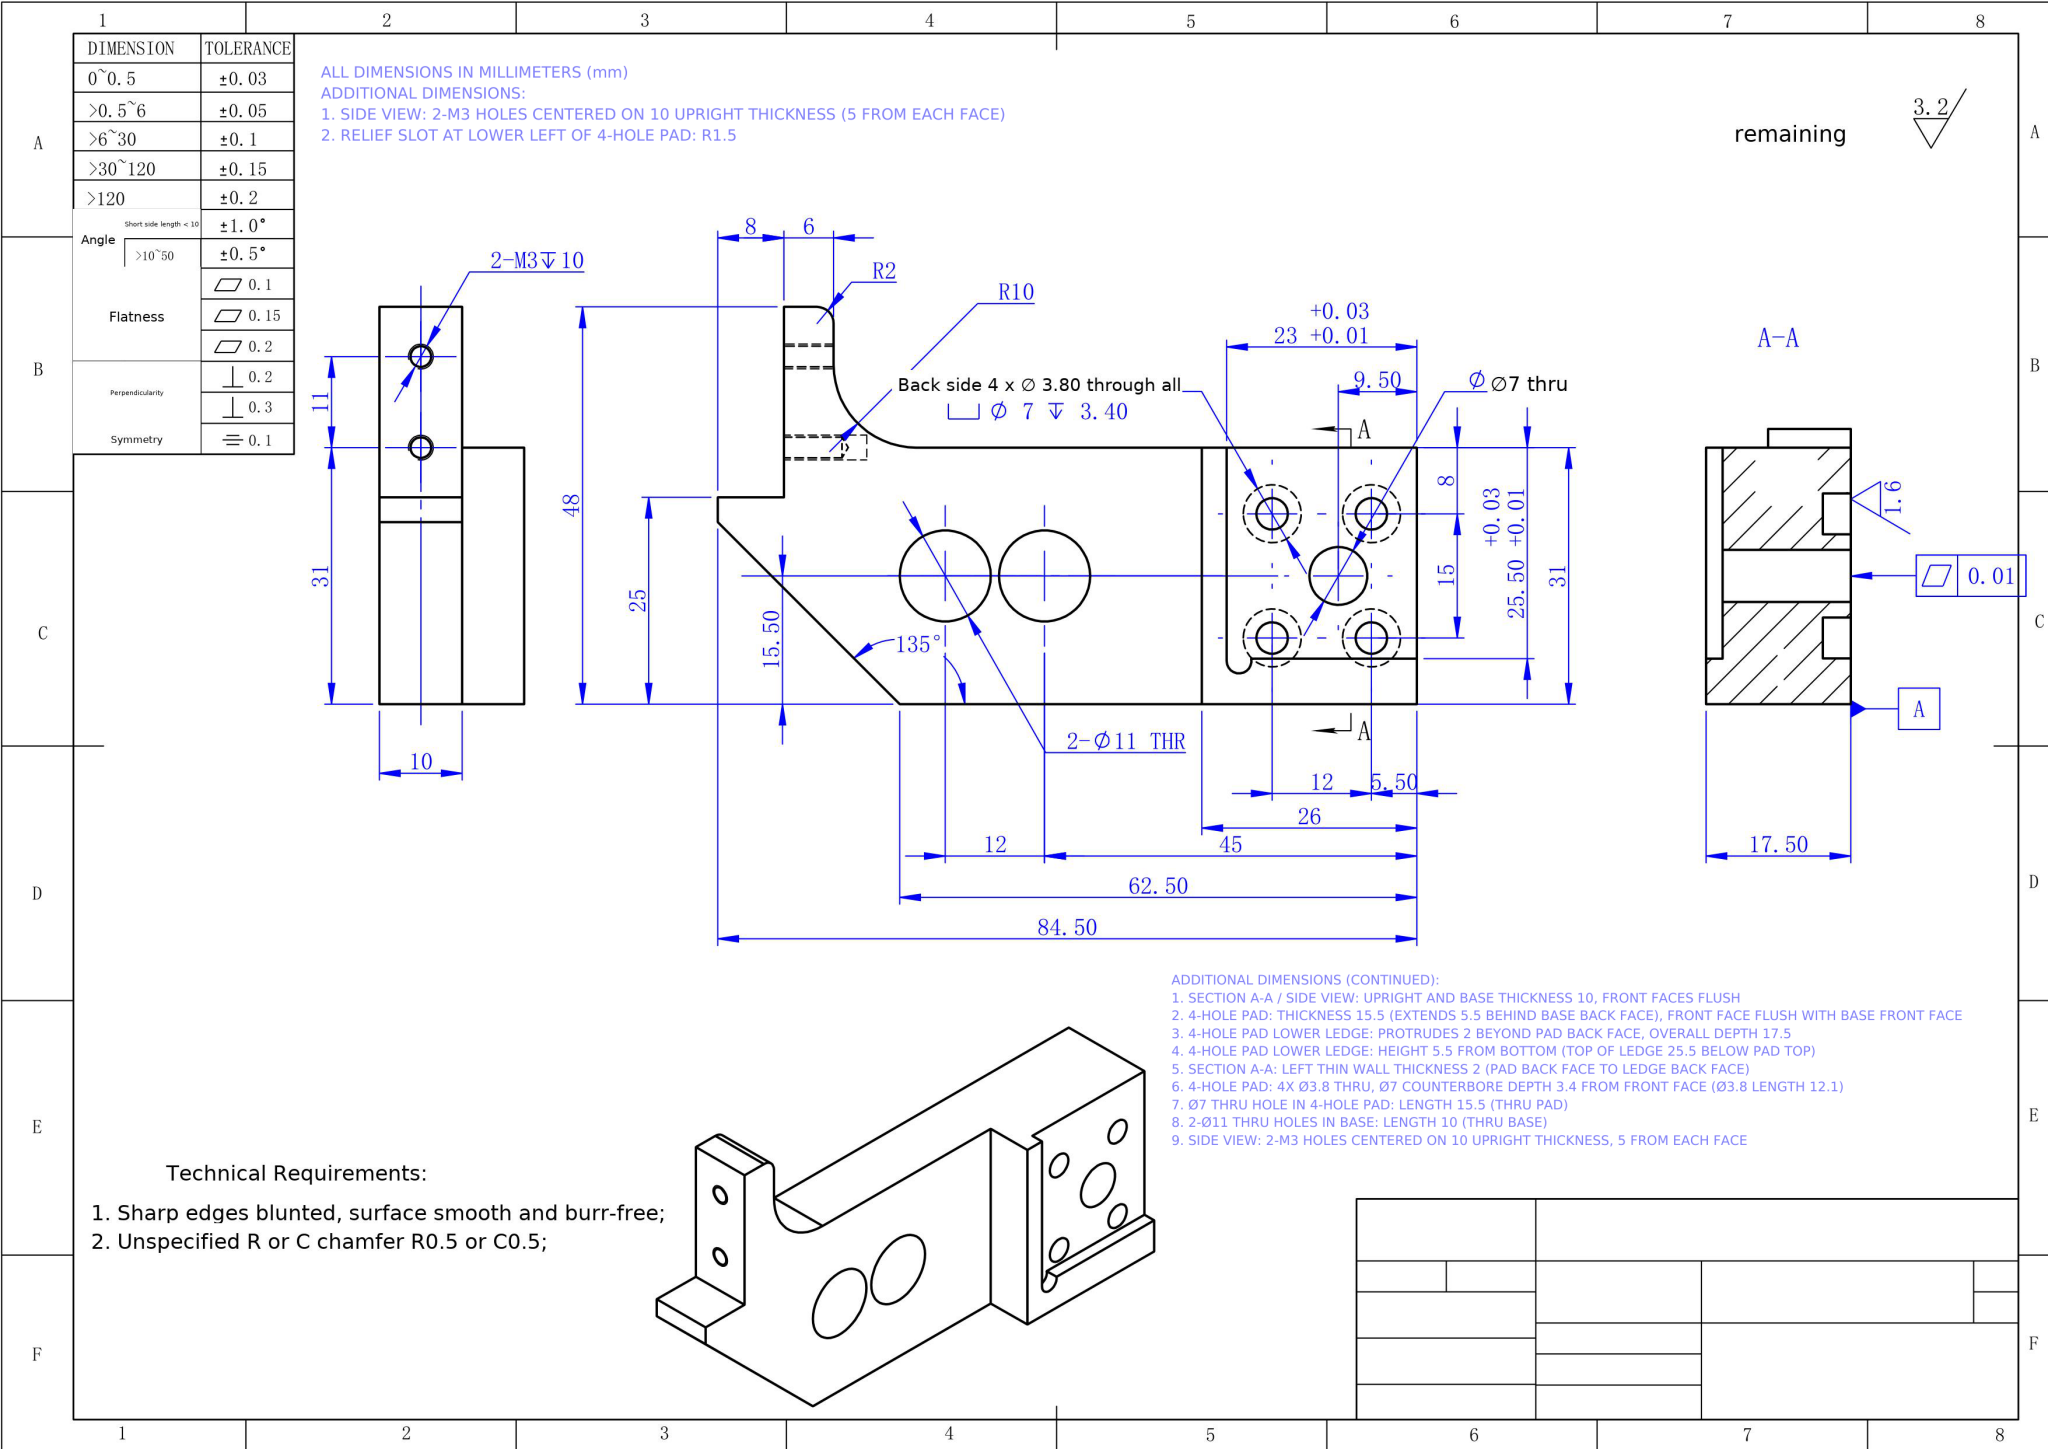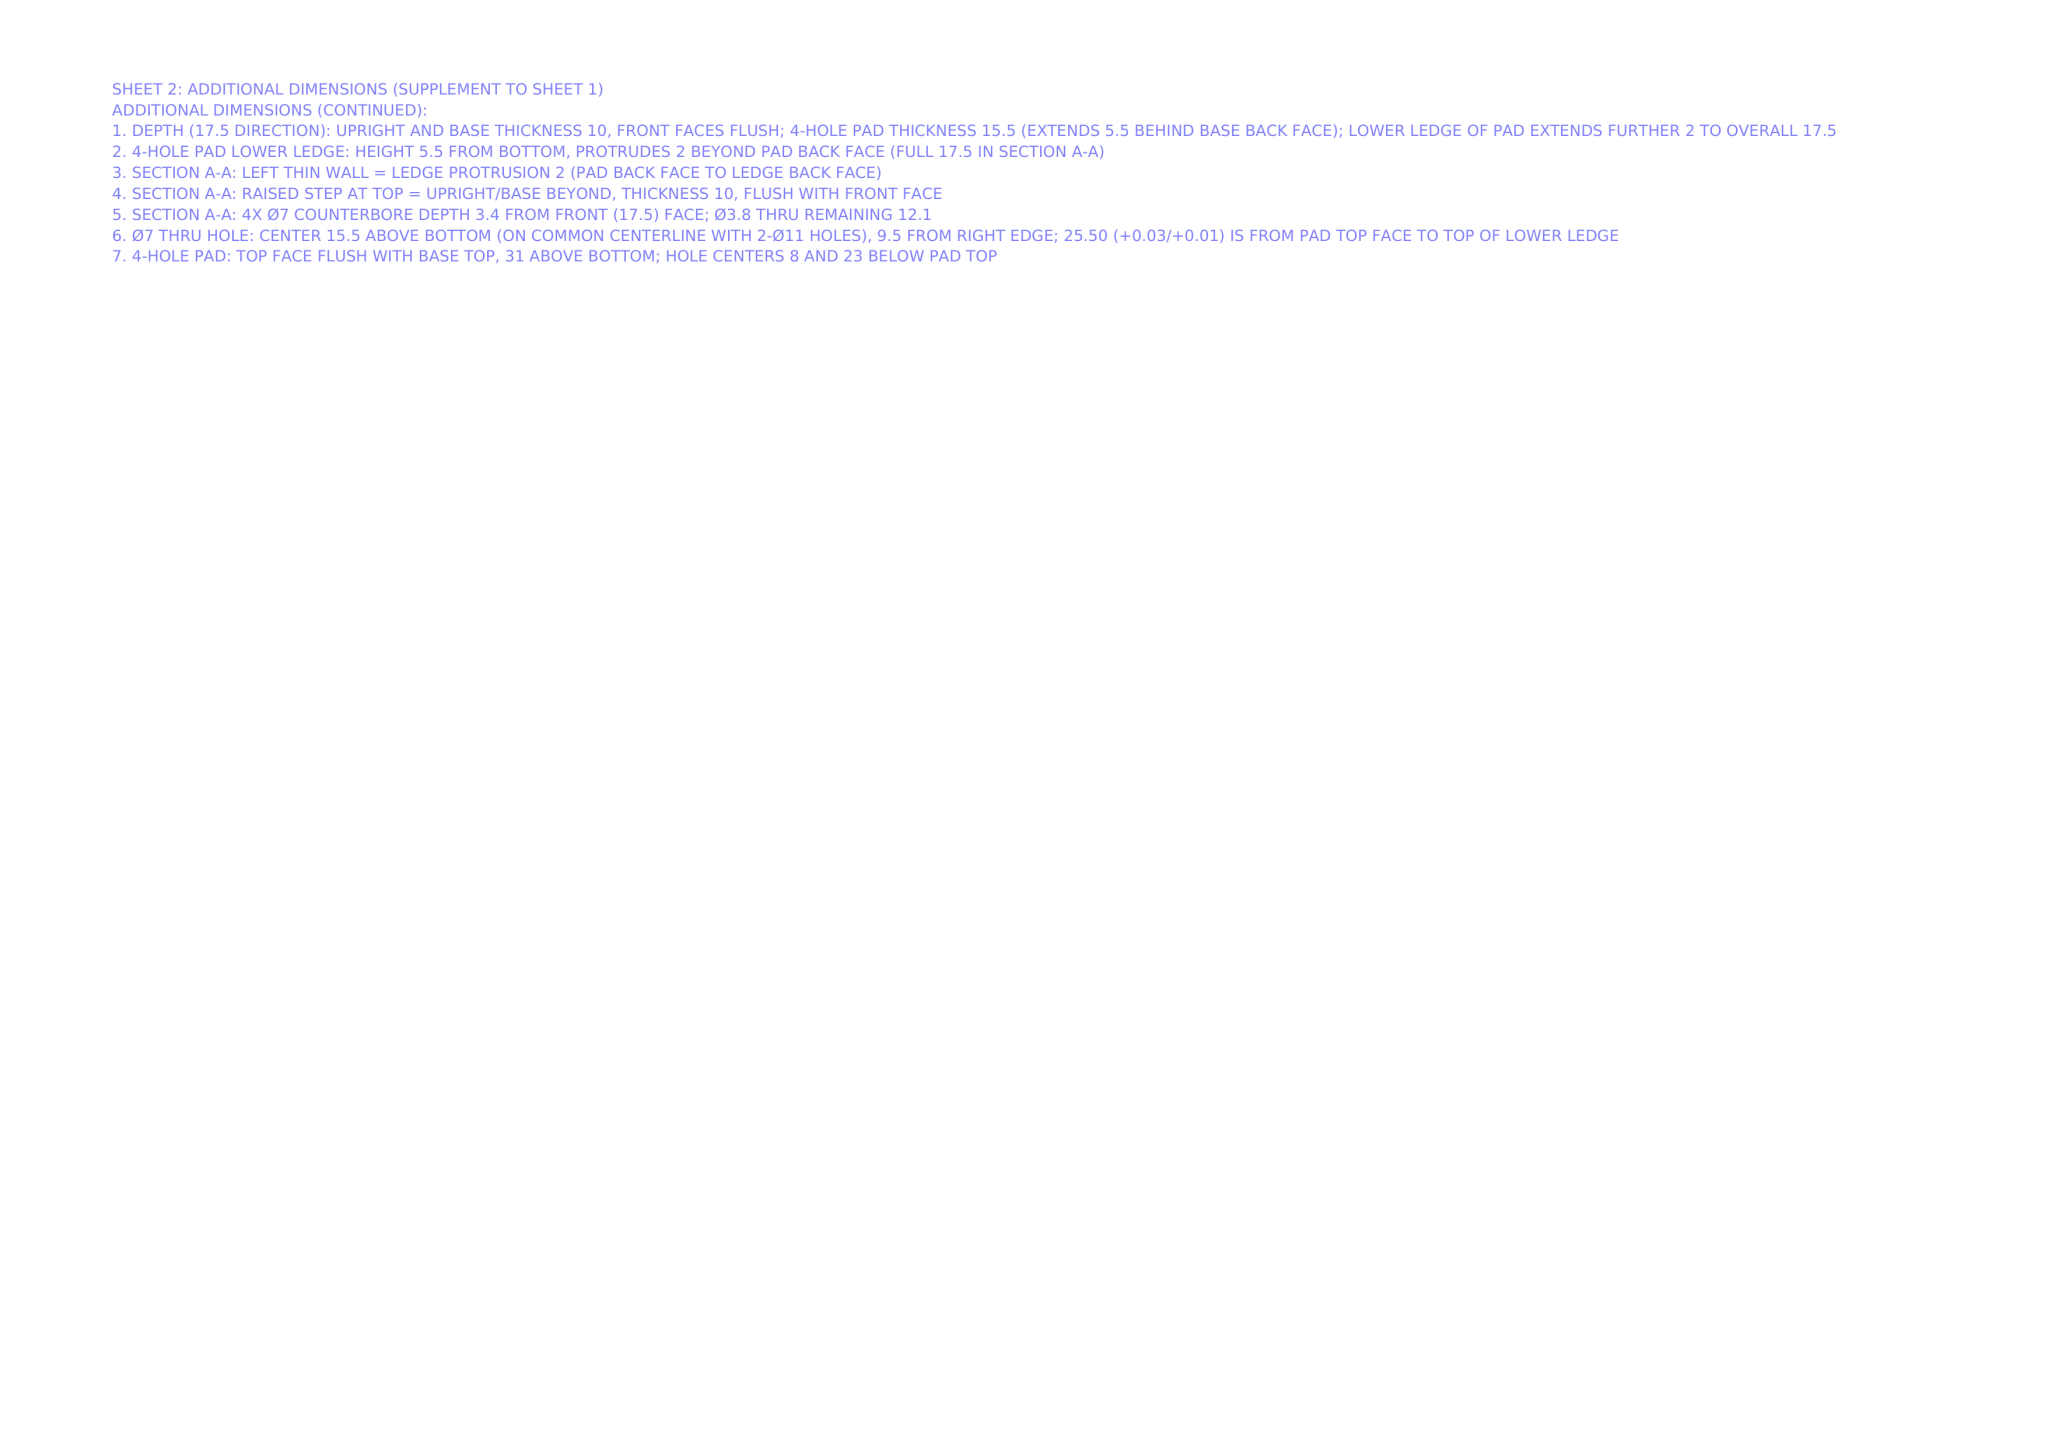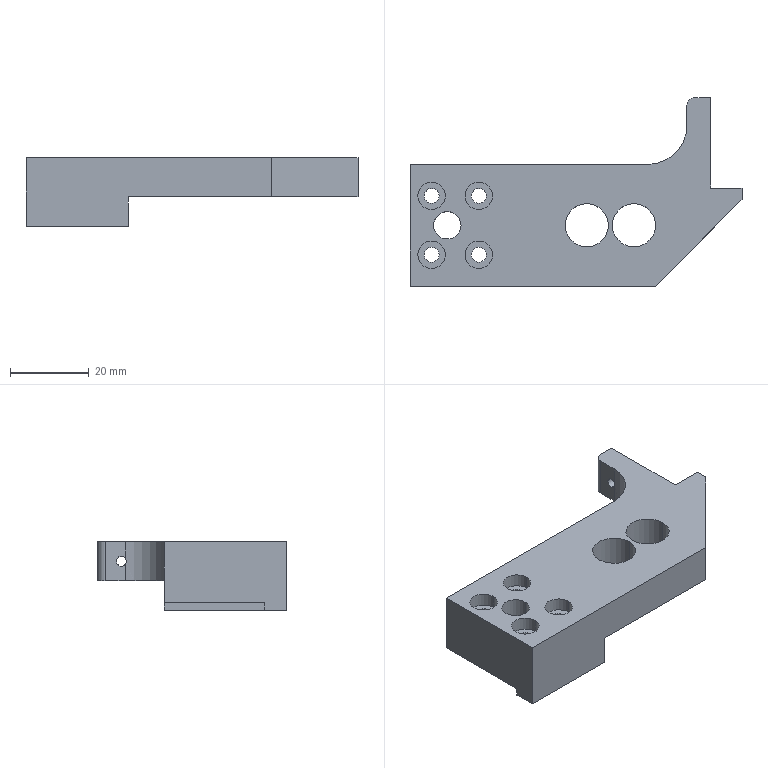Part | NX | mm | 1 solid | 51 faces | box 84.5 x 48 x 17.5 mm | volume 25750 mm3 | cylinder 29 | plane 20 | cone 2 | commonest cylinder face diameters 7 x10 3.8 x8 2.5 x4 11 x4 20 x1 4 x1 3 x1